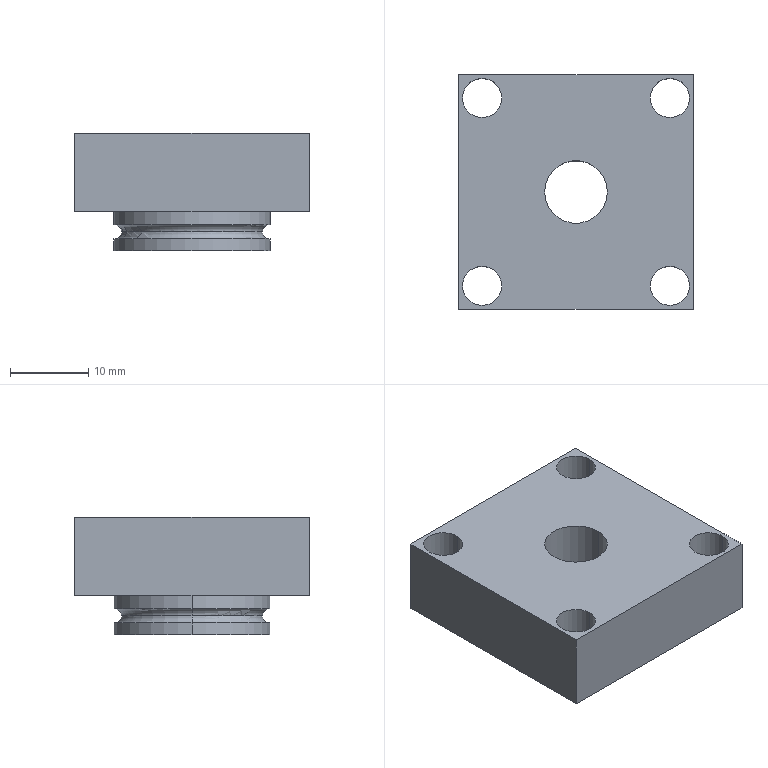Component | SolidWorks | FrontEndCapAssembly-1_CylinderFrontCover-1 | 1 solid | 25 faces | box 30 x 30 x 15 mm | volume 8944 mm3 | cylinder 14 | plane 7 | torus 4 | commonest cylinder face diameters 5 x8 20 x4 8 x2
build123d program:
from build123d import *

# Parameters (mm, degrees)
SKETCH1_W         = 30
SKETCH1_H         = 30
EXTRUDE1_DEPTH    = 10
SKETCH5_R         = 10
EXTRUDE5_DEPTH    = 5
SKETCH6_R         = 4
EXTRUDE6_DEPTH    = 30.059
SKETCH7_R         = 2.5
EXTRUDE7_DEPTH    = 30.059
CIRPATTERN1_COUNT = 4
SKETCH8_R         = 0.9


with BuildPart() as part:
    # Sketch1 → Extrude1 (new body)
    with BuildSketch(Plane.XY):
        with Locations((-3.842, -1.261)):
            Rectangle(SKETCH1_W, SKETCH1_H)
    extrude(amount=EXTRUDE1_DEPTH)

    # Sketch5 → Extrude5 (add)
    with BuildSketch(Plane.XY.offset(10)):
        with Locations((-3.842, -1.261)):
            Circle(SKETCH5_R)
    extrude(amount=EXTRUDE5_DEPTH)

    # Sketch6 → Extrude6 (cut, through all)
    with BuildSketch(Plane.XY.offset(15)):
        with Locations((-3.842, -1.261)):
            Circle(SKETCH6_R)
    extrude(amount=-EXTRUDE6_DEPTH, mode=Mode.SUBTRACT)

    # Sketch7 → Extrude7 (cut, through all)
    with BuildSketch(Plane(origin=(0, 0, 0), x_dir=(-1, 0, 0), z_dir=(0, 0, -1))):
        with Locations((-8.158, 10.739)):
            Circle(SKETCH7_R)
    extrude7 = extrude(amount=-EXTRUDE7_DEPTH, mode=Mode.SUBTRACT)

    # CirPattern1: Extrude7 ×4 about axis
    cirpattern1_axis = Axis((-3.842, -1.261, 0), (0, 0, 1))
    for i in range(1, CIRPATTERN1_COUNT):
        add(extrude7.rotate(cirpattern1_axis, i * 360 / CIRPATTERN1_COUNT), mode=Mode.SUBTRACT)

    # Sketch8 → Cut-Revolve1 (revolve, cut)
    with BuildSketch(Plane.ZY.offset(3.842), mode=Mode.PRIVATE) as cut_revolve1_sk:
        with Locations((12.6, 8.639)):
            Circle(SKETCH8_R)
    revolve(cut_revolve1_sk.sketch.rotate(Axis((-3.842, -1.261, 0), (0, 0, 1)), 90), axis=Axis((-3.842, -1.261, 0), (0, 0, 1)), mode=Mode.SUBTRACT)


solid = part.part

# Placed as in the assembly
solid = solid.moved(Location((9.967, -2.907, 52.5), (180, 0, 0)))
STEP:
#1=COLOUR_RGB('',0.7922,0.8196,0.9333);
#2=FILL_AREA_STYLE_COLOUR('',#1);
#3=FILL_AREA_STYLE('',(#2));
#4=SURFACE_STYLE_FILL_AREA(#3);
#5=SURFACE_SIDE_STYLE('',(#4));
#6=SURFACE_STYLE_USAGE(.BOTH.,#5);
#7=PRESENTATION_STYLE_ASSIGNMENT((#6));
#8=CARTESIAN_POINT('',(0.6348,-0.06482,1.606));
#9=VERTEX_POINT('',#8);
#10=CARTESIAN_POINT('',(0.5955,-0.06482,1.571));
#11=VERTEX_POINT('',#10);
#12=CARTESIAN_POINT('',(0.6309,-0.06482,1.571));
#13=DIRECTION('',(0.,-1.,-0.));
#14=DIRECTION('',(1.,0.,0.));
#15=AXIS2_PLACEMENT_3D('',#12,#13,#14);
#16=CIRCLE('',#15,0.03543);
#17=EDGE_CURVE('',#9,#11,#16,.T.);
#18=ORIENTED_EDGE('',*,*,#17,.T.);
#19=CARTESIAN_POINT('',(-0.1132,-0.06482,1.571));
#20=VERTEX_POINT('',#19);
#21=CARTESIAN_POINT('',(0.2411,-0.06482,1.571));
#22=DIRECTION('',(-0.,-0.,1.));
#23=DIRECTION('',(1.,0.,0.));
#24=AXIS2_PLACEMENT_3D('',#21,#22,#23);
#25=CIRCLE('',#24,0.3543);
#26=EDGE_CURVE('',#11,#20,#25,.T.);
#27=ORIENTED_EDGE('',*,*,#26,.T.);
#28=CARTESIAN_POINT('',(-0.1526,-0.06482,1.606));
#29=VERTEX_POINT('',#28);
#30=CARTESIAN_POINT('',(-0.1486,-0.06482,1.571));
#31=DIRECTION('',(-0.,1.,0.));
#32=DIRECTION('',(-1.,-0.,0.));
#33=AXIS2_PLACEMENT_3D('',#30,#31,#32);
#34=CIRCLE('',#33,0.03543);
#35=EDGE_CURVE('',#29,#20,#34,.T.);
#36=ORIENTED_EDGE('',*,*,#35,.F.);
#37=CARTESIAN_POINT('',(0.2411,-0.06482,1.606));
#38=DIRECTION('',(0.,0.,-1.));
#39=DIRECTION('',(-1.,-0.,0.));
#40=AXIS2_PLACEMENT_3D('',#37,#38,#39);
#41=CIRCLE('',#40,0.3937);
#42=EDGE_CURVE('',#29,#9,#41,.T.);
#43=ORIENTED_EDGE('',*,*,#42,.T.);
#44=EDGE_LOOP('',(#18,#27,#36,#43));
#45=FACE_OUTER_BOUND('',#44,.T.);
#46=CARTESIAN_POINT('',(0.2411,-0.06482,1.571));
#47=DIRECTION('',(-0.,-0.,1.));
#48=DIRECTION('',(1.,0.,0.));
#49=AXIS2_PLACEMENT_3D('',#46,#47,#48);
#50=TOROIDAL_SURFACE('',#49,0.3898,0.03543);
#51=ADVANCED_FACE('',(#45),#50,.F.);
#52=ORIENTED_EDGE('',*,*,#35,.T.);
#53=CARTESIAN_POINT('',(0.2411,-0.06482,1.571));
#54=DIRECTION('',(-0.,-0.,1.));
#55=DIRECTION('',(1.,0.,0.));
#56=AXIS2_PLACEMENT_3D('',#53,#54,#55);
#57=CIRCLE('',#56,0.3543);
#58=EDGE_CURVE('',#20,#11,#57,.T.);
#59=ORIENTED_EDGE('',*,*,#58,.T.);
#60=ORIENTED_EDGE('',*,*,#17,.F.);
#61=CARTESIAN_POINT('',(0.2411,-0.06482,1.606));
#62=DIRECTION('',(0.,0.,-1.));
#63=DIRECTION('',(-1.,-0.,0.));
#64=AXIS2_PLACEMENT_3D('',#61,#62,#63);
#65=CIRCLE('',#64,0.3937);
#66=EDGE_CURVE('',#9,#29,#65,.T.);
#67=ORIENTED_EDGE('',*,*,#66,.T.);
#68=EDGE_LOOP('',(#52,#59,#60,#67));
#69=FACE_OUTER_BOUND('',#68,.T.);
#70=CARTESIAN_POINT('',(0.2411,-0.06482,1.571));
#71=DIRECTION('',(-0.,-0.,1.));
#72=DIRECTION('',(1.,0.,0.));
#73=AXIS2_PLACEMENT_3D('',#70,#71,#72);
#74=TOROIDAL_SURFACE('',#73,0.3898,0.03543);
#75=ADVANCED_FACE('',(#69),#74,.F.);
#76=ORIENTED_EDGE('',*,*,#58,.F.);
#77=CARTESIAN_POINT('',(-0.1526,-0.06482,1.536));
#78=VERTEX_POINT('',#77);
#79=CARTESIAN_POINT('',(-0.1486,-0.06482,1.571));
#80=DIRECTION('',(-0.,1.,0.));
#81=DIRECTION('',(-1.,-0.,0.));
#82=AXIS2_PLACEMENT_3D('',#79,#80,#81);
#83=CIRCLE('',#82,0.03543);
#84=EDGE_CURVE('',#20,#78,#83,.T.);
#85=ORIENTED_EDGE('',*,*,#84,.T.);
#86=CARTESIAN_POINT('',(0.6348,-0.06482,1.536));
#87=VERTEX_POINT('',#86);
#88=CARTESIAN_POINT('',(0.2411,-0.06482,1.536));
#89=DIRECTION('',(-0.,-0.,1.));
#90=DIRECTION('',(1.,0.,0.));
#91=AXIS2_PLACEMENT_3D('',#88,#89,#90);
#92=CIRCLE('',#91,0.3937);
#93=EDGE_CURVE('',#78,#87,#92,.T.);
#94=ORIENTED_EDGE('',*,*,#93,.T.);
#95=CARTESIAN_POINT('',(0.6309,-0.06482,1.571));
#96=DIRECTION('',(0.,-1.,-0.));
#97=DIRECTION('',(1.,0.,0.));
#98=AXIS2_PLACEMENT_3D('',#95,#96,#97);
#99=CIRCLE('',#98,0.03543);
#100=EDGE_CURVE('',#11,#87,#99,.T.);
#101=ORIENTED_EDGE('',*,*,#100,.F.);
#102=EDGE_LOOP('',(#76,#85,#94,#101));
#103=FACE_OUTER_BOUND('',#102,.T.);
#104=CARTESIAN_POINT('',(0.2411,-0.06482,1.571));
#105=DIRECTION('',(-0.,-0.,1.));
#106=DIRECTION('',(1.,0.,0.));
#107=AXIS2_PLACEMENT_3D('',#104,#105,#106);
#108=TOROIDAL_SURFACE('',#107,0.3898,0.03543);
#109=ADVANCED_FACE('',(#103),#108,.F.);
#110=CARTESIAN_POINT('',(-0.1329,-0.5373,1.673));
#111=VERTEX_POINT('',#110);
#112=CARTESIAN_POINT('',(-0.3297,-0.5373,1.673));
#113=VERTEX_POINT('',#112);
#114=CARTESIAN_POINT('',(-0.2313,-0.5373,1.673));
#115=DIRECTION('',(0.,0.,-1.));
#116=DIRECTION('',(-1.,-0.,0.));
#117=AXIS2_PLACEMENT_3D('',#114,#115,#116);
#118=CIRCLE('',#117,0.09843);
#119=EDGE_CURVE('',#111,#113,#118,.T.);
#120=ORIENTED_EDGE('',*,*,#119,.T.);
#121=CARTESIAN_POINT('',(-0.3297,-0.5373,2.067));
#122=VERTEX_POINT('',#121);
#123=CARTESIAN_POINT('',(-0.3297,-0.5373,1.476));
#124=DIRECTION('',(-0.,-0.,1.));
#125=VECTOR('',#124,39.37);
#126=LINE('',#123,#125);
#127=EDGE_CURVE('',#113,#122,#126,.T.);
#128=ORIENTED_EDGE('',*,*,#127,.T.);
#129=CARTESIAN_POINT('',(-0.1329,-0.5373,2.067));
#130=VERTEX_POINT('',#129);
#131=CARTESIAN_POINT('',(-0.2313,-0.5373,2.067));
#132=DIRECTION('',(-0.,-0.,1.));
#133=DIRECTION('',(0.,1.,0.));
#134=AXIS2_PLACEMENT_3D('',#131,#132,#133);
#135=CIRCLE('',#134,0.09843);
#136=EDGE_CURVE('',#122,#130,#135,.T.);
#137=ORIENTED_EDGE('',*,*,#136,.T.);
#138=CARTESIAN_POINT('',(-0.1329,-0.5373,1.476));
#139=DIRECTION('',(-0.,-0.,1.));
#140=VECTOR('',#139,39.37);
#141=LINE('',#138,#140);
#142=EDGE_CURVE('',#111,#130,#141,.T.);
#143=ORIENTED_EDGE('',*,*,#142,.F.);
#144=EDGE_LOOP('',(#120,#128,#137,#143));
#145=FACE_OUTER_BOUND('',#144,.T.);
#146=CARTESIAN_POINT('',(-0.2313,-0.5373,1.476));
#147=DIRECTION('',(-0.,-0.,1.));
#148=DIRECTION('',(1.,0.,0.));
#149=AXIS2_PLACEMENT_3D('',#146,#147,#148);
#150=CYLINDRICAL_SURFACE('',#149,0.09843);
#151=ADVANCED_FACE('',(#145),#150,.F.);
#152=CARTESIAN_POINT('',(0.812,-0.5373,1.673));
#153=VERTEX_POINT('',#152);
#154=CARTESIAN_POINT('',(0.6152,-0.5373,1.673));
#155=VERTEX_POINT('',#154);
#156=CARTESIAN_POINT('',(0.7136,-0.5373,1.673));
#157=DIRECTION('',(0.,0.,-1.));
#158=DIRECTION('',(-1.,-0.,0.));
#159=AXIS2_PLACEMENT_3D('',#156,#157,#158);
#160=CIRCLE('',#159,0.09843);
#161=EDGE_CURVE('',#153,#155,#160,.T.);
#162=ORIENTED_EDGE('',*,*,#161,.T.);
#163=CARTESIAN_POINT('',(0.6152,-0.5373,2.067));
#164=VERTEX_POINT('',#163);
#165=CARTESIAN_POINT('',(0.6152,-0.5373,1.476));
#166=DIRECTION('',(-0.,-0.,1.));
#167=VECTOR('',#166,39.37);
#168=LINE('',#165,#167);
#169=EDGE_CURVE('',#155,#164,#168,.T.);
#170=ORIENTED_EDGE('',*,*,#169,.T.);
#171=CARTESIAN_POINT('',(0.812,-0.5373,2.067));
#172=VERTEX_POINT('',#171);
#173=CARTESIAN_POINT('',(0.7136,-0.5373,2.067));
#174=DIRECTION('',(-0.,-0.,1.));
#175=DIRECTION('',(-1.,0.,0.));
#176=AXIS2_PLACEMENT_3D('',#173,#174,#175);
#177=CIRCLE('',#176,0.09843);
#178=EDGE_CURVE('',#164,#172,#177,.T.);
#179=ORIENTED_EDGE('',*,*,#178,.T.);
#180=CARTESIAN_POINT('',(0.812,-0.5373,1.476));
#181=DIRECTION('',(-0.,-0.,1.));
#182=VECTOR('',#181,39.37);
#183=LINE('',#180,#182);
#184=EDGE_CURVE('',#153,#172,#183,.T.);
#185=ORIENTED_EDGE('',*,*,#184,.F.);
#186=EDGE_LOOP('',(#162,#170,#179,#185));
#187=FACE_OUTER_BOUND('',#186,.T.);
#188=CARTESIAN_POINT('',(0.7136,-0.5373,1.476));
#189=DIRECTION('',(-0.,-0.,1.));
#190=DIRECTION('',(1.,0.,0.));
#191=AXIS2_PLACEMENT_3D('',#188,#189,#190);
#192=CYLINDRICAL_SURFACE('',#191,0.09843);
#193=ADVANCED_FACE('',(#187),#192,.F.);
#194=CARTESIAN_POINT('',(0.812,0.4076,1.673));
#195=VERTEX_POINT('',#194);
#196=CARTESIAN_POINT('',(0.6152,0.4076,1.673));
#197=VERTEX_POINT('',#196);
#198=CARTESIAN_POINT('',(0.7136,0.4076,1.673));
#199=DIRECTION('',(0.,0.,-1.));
#200=DIRECTION('',(-1.,-0.,0.));
#201=AXIS2_PLACEMENT_3D('',#198,#199,#200);
#202=CIRCLE('',#201,0.09843);
#203=EDGE_CURVE('',#195,#197,#202,.T.);
#204=ORIENTED_EDGE('',*,*,#203,.T.);
#205=CARTESIAN_POINT('',(0.6152,0.4076,2.067));
#206=VERTEX_POINT('',#205);
#207=CARTESIAN_POINT('',(0.6152,0.4076,1.476));
#208=DIRECTION('',(-0.,-0.,1.));
#209=VECTOR('',#208,39.37);
#210=LINE('',#207,#209);
#211=EDGE_CURVE('',#197,#206,#210,.T.);
#212=ORIENTED_EDGE('',*,*,#211,.T.);
#213=CARTESIAN_POINT('',(0.812,0.4076,2.067));
#214=VERTEX_POINT('',#213);
#215=CARTESIAN_POINT('',(0.7136,0.4076,2.067));
#216=DIRECTION('',(-0.,-0.,1.));
#217=DIRECTION('',(-0.,-1.,0.));
#218=AXIS2_PLACEMENT_3D('',#215,#216,#217);
#219=CIRCLE('',#218,0.09843);
#220=EDGE_CURVE('',#206,#214,#219,.T.);
#221=ORIENTED_EDGE('',*,*,#220,.T.);
#222=CARTESIAN_POINT('',(0.812,0.4076,1.476));
#223=DIRECTION('',(-0.,-0.,1.));
#224=VECTOR('',#223,39.37);
#225=LINE('',#222,#224);
#226=EDGE_CURVE('',#195,#214,#225,.T.);
#227=ORIENTED_EDGE('',*,*,#226,.F.);
#228=EDGE_LOOP('',(#204,#212,#221,#227));
#229=FACE_OUTER_BOUND('',#228,.T.);
#230=CARTESIAN_POINT('',(0.7136,0.4076,1.476));
#231=DIRECTION('',(-0.,-0.,1.));
#232=DIRECTION('',(1.,0.,0.));
#233=AXIS2_PLACEMENT_3D('',#230,#231,#232);
#234=CYLINDRICAL_SURFACE('',#233,0.09843);
#235=ADVANCED_FACE('',(#229),#234,.F.);
#236=CARTESIAN_POINT('',(-0.1329,0.4076,1.673));
#237=VERTEX_POINT('',#236);
#238=CARTESIAN_POINT('',(-0.3297,0.4076,1.673));
#239=VERTEX_POINT('',#238);
#240=CARTESIAN_POINT('',(-0.2313,0.4076,1.673));
#241=DIRECTION('',(0.,0.,-1.));
#242=DIRECTION('',(-1.,-0.,0.));
#243=AXIS2_PLACEMENT_3D('',#240,#241,#242);
#244=CIRCLE('',#243,0.09843);
#245=EDGE_CURVE('',#237,#239,#244,.T.);
#246=ORIENTED_EDGE('',*,*,#245,.T.);
#247=CARTESIAN_POINT('',(-0.3297,0.4076,2.067));
#248=VERTEX_POINT('',#247);
#249=CARTESIAN_POINT('',(-0.3297,0.4076,1.476));
#250=DIRECTION('',(-0.,-0.,1.));
#251=VECTOR('',#250,39.37);
#252=LINE('',#249,#251);
#253=EDGE_CURVE('',#239,#248,#252,.T.);
#254=ORIENTED_EDGE('',*,*,#253,.T.);
#255=CARTESIAN_POINT('',(-0.1329,0.4076,2.067));
#256=VERTEX_POINT('',#255);
#257=CARTESIAN_POINT('',(-0.2313,0.4076,2.067));
#258=DIRECTION('',(-0.,-0.,1.));
#259=DIRECTION('',(1.,0.,0.));
#260=AXIS2_PLACEMENT_3D('',#257,#258,#259);
#261=CIRCLE('',#260,0.09843);
#262=EDGE_CURVE('',#248,#256,#261,.T.);
#263=ORIENTED_EDGE('',*,*,#262,.T.);
#264=CARTESIAN_POINT('',(-0.1329,0.4076,1.476));
#265=DIRECTION('',(-0.,-0.,1.));
#266=VECTOR('',#265,39.37);
#267=LINE('',#264,#266);
#268=EDGE_CURVE('',#237,#256,#267,.T.);
#269=ORIENTED_EDGE('',*,*,#268,.F.);
#270=EDGE_LOOP('',(#246,#254,#263,#269));
#271=FACE_OUTER_BOUND('',#270,.T.);
#272=CARTESIAN_POINT('',(-0.2313,0.4076,1.476));
#273=DIRECTION('',(-0.,-0.,1.));
#274=DIRECTION('',(1.,0.,0.));
#275=AXIS2_PLACEMENT_3D('',#272,#273,#274);
#276=CYLINDRICAL_SURFACE('',#275,0.09843);
#277=ADVANCED_FACE('',(#271),#276,.F.);
#278=CARTESIAN_POINT('',(0.3986,-0.06482,2.067));
#279=VERTEX_POINT('',#278);
#280=CARTESIAN_POINT('',(0.08366,-0.06482,2.067));
#281=VERTEX_POINT('',#280);
#282=CARTESIAN_POINT('',(0.2411,-0.06482,2.067));
#283=DIRECTION('',(0.,0.,-1.));
#284=DIRECTION('',(-1.,-0.,0.));
#285=AXIS2_PLACEMENT_3D('',#282,#283,#284);
#286=CIRCLE('',#285,0.1575);
#287=EDGE_CURVE('',#279,#281,#286,.T.);
#288=ORIENTED_EDGE('',*,*,#287,.F.);
#289=CARTESIAN_POINT('',(0.3986,-0.06482,1.476));
#290=VERTEX_POINT('',#289);
#291=CARTESIAN_POINT('',(0.3986,-0.06482,2.067));
#292=DIRECTION('',(0.,0.,-1.));
#293=VECTOR('',#292,39.37);
#294=LINE('',#291,#293);
#295=EDGE_CURVE('',#279,#290,#294,.T.);
#296=ORIENTED_EDGE('',*,*,#295,.T.);
#297=CARTESIAN_POINT('',(0.08366,-0.06482,1.476));
#298=VERTEX_POINT('',#297);
#299=CARTESIAN_POINT('',(0.2411,-0.06482,1.476));
#300=DIRECTION('',(0.,0.,-1.));
#301=DIRECTION('',(-1.,-0.,0.));
#302=AXIS2_PLACEMENT_3D('',#299,#300,#301);
#303=CIRCLE('',#302,0.1575);
#304=EDGE_CURVE('',#290,#298,#303,.T.);
#305=ORIENTED_EDGE('',*,*,#304,.T.);
#306=CARTESIAN_POINT('',(0.08366,-0.06482,2.067));
#307=DIRECTION('',(0.,0.,-1.));
#308=VECTOR('',#307,39.37);
#309=LINE('',#306,#308);
#310=EDGE_CURVE('',#281,#298,#309,.T.);
#311=ORIENTED_EDGE('',*,*,#310,.F.);
#312=EDGE_LOOP('',(#288,#296,#305,#311));
#313=FACE_OUTER_BOUND('',#312,.T.);
#314=CARTESIAN_POINT('',(0.2411,-0.06482,2.067));
#315=DIRECTION('',(0.,0.,-1.));
#316=DIRECTION('',(-1.,-0.,0.));
#317=AXIS2_PLACEMENT_3D('',#314,#315,#316);
#318=CYLINDRICAL_SURFACE('',#317,0.1575);
#319=ADVANCED_FACE('',(#313),#318,.F.);
#320=CARTESIAN_POINT('',(-0.1526,-0.06482,1.476));
#321=VERTEX_POINT('',#320);
#322=CARTESIAN_POINT('',(0.6348,-0.06482,1.476));
#323=VERTEX_POINT('',#322);
#324=CARTESIAN_POINT('',(0.2411,-0.06482,1.476));
#325=DIRECTION('',(0.,0.,-1.));
#326=DIRECTION('',(-1.,-0.,0.));
#327=AXIS2_PLACEMENT_3D('',#324,#325,#326);
#328=CIRCLE('',#327,0.3937);
#329=EDGE_CURVE('',#321,#323,#328,.T.);
#330=ORIENTED_EDGE('',*,*,#329,.F.);
#331=CARTESIAN_POINT('',(-0.1526,-0.06482,1.476));
#332=DIRECTION('',(-0.,-0.,1.));
#333=VECTOR('',#332,39.37);
#334=LINE('',#331,#333);
#335=EDGE_CURVE('',#321,#78,#334,.T.);
#336=ORIENTED_EDGE('',*,*,#335,.T.);
#337=CARTESIAN_POINT('',(0.2411,-0.06482,1.536));
#338=DIRECTION('',(-0.,-0.,1.));
#339=DIRECTION('',(1.,0.,0.));
#340=AXIS2_PLACEMENT_3D('',#337,#338,#339);
#341=CIRCLE('',#340,0.3937);
#342=EDGE_CURVE('',#87,#78,#341,.T.);
#343=ORIENTED_EDGE('',*,*,#342,.F.);
#344=CARTESIAN_POINT('',(0.6348,-0.06482,1.476));
#345=DIRECTION('',(-0.,-0.,1.));
#346=VECTOR('',#345,39.37);
#347=LINE('',#344,#346);
#348=EDGE_CURVE('',#323,#87,#347,.T.);
#349=ORIENTED_EDGE('',*,*,#348,.F.);
#350=EDGE_LOOP('',(#330,#336,#343,#349));
#351=FACE_OUTER_BOUND('',#350,.T.);
#352=CARTESIAN_POINT('',(0.2411,-0.06482,1.476));
#353=DIRECTION('',(-0.,-0.,1.));
#354=DIRECTION('',(1.,0.,0.));
#355=AXIS2_PLACEMENT_3D('',#352,#353,#354);
#356=CYLINDRICAL_SURFACE('',#355,0.3937);
#357=ADVANCED_FACE('',(#351),#356,.T.);
#358=ORIENTED_EDGE('',*,*,#42,.F.);
#359=CARTESIAN_POINT('',(-0.1526,-0.06482,1.673));
#360=VERTEX_POINT('',#359);
#361=CARTESIAN_POINT('',(-0.1526,-0.06482,1.476));
#362=DIRECTION('',(-0.,-0.,1.));
#363=VECTOR('',#362,39.37);
#364=LINE('',#361,#363);
#365=EDGE_CURVE('',#29,#360,#364,.T.);
#366=ORIENTED_EDGE('',*,*,#365,.T.);
#367=CARTESIAN_POINT('',(0.6348,-0.06482,1.673));
#368=VERTEX_POINT('',#367);
#369=CARTESIAN_POINT('',(0.2411,-0.06482,1.673));
#370=DIRECTION('',(0.,0.,-1.));
#371=DIRECTION('',(-1.,-0.,0.));
#372=AXIS2_PLACEMENT_3D('',#369,#370,#371);
#373=CIRCLE('',#372,0.3937);
#374=EDGE_CURVE('',#360,#368,#373,.T.);
#375=ORIENTED_EDGE('',*,*,#374,.T.);
#376=CARTESIAN_POINT('',(0.6348,-0.06482,1.476));
#377=DIRECTION('',(-0.,-0.,1.));
#378=VECTOR('',#377,39.37);
#379=LINE('',#376,#378);
#380=EDGE_CURVE('',#9,#368,#379,.T.);
#381=ORIENTED_EDGE('',*,*,#380,.F.);
#382=EDGE_LOOP('',(#358,#366,#375,#381));
#383=FACE_OUTER_BOUND('',#382,.T.);
#384=CARTESIAN_POINT('',(0.2411,-0.06482,1.476));
#385=DIRECTION('',(-0.,-0.,1.));
#386=DIRECTION('',(1.,0.,0.));
#387=AXIS2_PLACEMENT_3D('',#384,#385,#386);
#388=CYLINDRICAL_SURFACE('',#387,0.3937);
#389=ADVANCED_FACE('',(#383),#388,.T.);
#390=ORIENTED_EDGE('',*,*,#365,.F.);
#391=ORIENTED_EDGE('',*,*,#66,.F.);
#392=ORIENTED_EDGE('',*,*,#380,.T.);
#393=CARTESIAN_POINT('',(0.2411,-0.06482,1.673));
#394=DIRECTION('',(0.,0.,-1.));
#395=DIRECTION('',(-1.,-0.,0.));
#396=AXIS2_PLACEMENT_3D('',#393,#394,#395);
#397=CIRCLE('',#396,0.3937);
#398=EDGE_CURVE('',#368,#360,#397,.T.);
#399=ORIENTED_EDGE('',*,*,#398,.T.);
#400=EDGE_LOOP('',(#390,#391,#392,#399));
#401=FACE_OUTER_BOUND('',#400,.T.);
#402=CARTESIAN_POINT('',(0.2411,-0.06482,1.476));
#403=DIRECTION('',(-0.,-0.,1.));
#404=DIRECTION('',(1.,0.,0.));
#405=AXIS2_PLACEMENT_3D('',#402,#403,#404);
#406=CYLINDRICAL_SURFACE('',#405,0.3937);
#407=ADVANCED_FACE('',(#401),#406,.T.);
#408=ORIENTED_EDGE('',*,*,#335,.F.);
#409=CARTESIAN_POINT('',(0.2411,-0.06482,1.476));
#410=DIRECTION('',(0.,0.,-1.));
#411=DIRECTION('',(-1.,-0.,0.));
#412=AXIS2_PLACEMENT_3D('',#409,#410,#411);
#413=CIRCLE('',#412,0.3937);
#414=EDGE_CURVE('',#323,#321,#413,.T.);
#415=ORIENTED_EDGE('',*,*,#414,.F.);
#416=ORIENTED_EDGE('',*,*,#348,.T.);
#417=ORIENTED_EDGE('',*,*,#93,.F.);
#418=EDGE_LOOP('',(#408,#415,#416,#417));
#419=FACE_OUTER_BOUND('',#418,.T.);
#420=CARTESIAN_POINT('',(0.2411,-0.06482,1.476));
#421=DIRECTION('',(-0.,-0.,1.));
#422=DIRECTION('',(1.,0.,0.));
#423=AXIS2_PLACEMENT_3D('',#420,#421,#422);
#424=CYLINDRICAL_SURFACE('',#423,0.3937);
#425=ADVANCED_FACE('',(#419),#424,.T.);
#426=ORIENTED_EDGE('',*,*,#119,.F.);
#427=CARTESIAN_POINT('',(-0.2313,-0.5373,1.673));
#428=DIRECTION('',(0.,0.,-1.));
#429=DIRECTION('',(-1.,-0.,0.));
#430=AXIS2_PLACEMENT_3D('',#427,#428,#429);
#431=CIRCLE('',#430,0.09843);
#432=EDGE_CURVE('',#113,#111,#431,.T.);
#433=ORIENTED_EDGE('',*,*,#432,.F.);
#434=EDGE_LOOP('',(#426,#433));
#435=FACE_BOUND('',#434,.T.);
#436=ORIENTED_EDGE('',*,*,#161,.F.);
#437=CARTESIAN_POINT('',(0.7136,-0.5373,1.673));
#438=DIRECTION('',(0.,0.,-1.));
#439=DIRECTION('',(-1.,-0.,0.));
#440=AXIS2_PLACEMENT_3D('',#437,#438,#439);
#441=CIRCLE('',#440,0.09843);
#442=EDGE_CURVE('',#155,#153,#441,.T.);
#443=ORIENTED_EDGE('',*,*,#442,.F.);
#444=EDGE_LOOP('',(#436,#443));
#445=FACE_BOUND('',#444,.T.);
#446=ORIENTED_EDGE('',*,*,#203,.F.);
#447=CARTESIAN_POINT('',(0.7136,0.4076,1.673));
#448=DIRECTION('',(0.,0.,-1.));
#449=DIRECTION('',(-1.,-0.,0.));
#450=AXIS2_PLACEMENT_3D('',#447,#448,#449);
#451=CIRCLE('',#450,0.09843);
#452=EDGE_CURVE('',#197,#195,#451,.T.);
#453=ORIENTED_EDGE('',*,*,#452,.F.);
#454=EDGE_LOOP('',(#446,#453));
#455=FACE_BOUND('',#454,.T.);
#456=ORIENTED_EDGE('',*,*,#245,.F.);
#457=CARTESIAN_POINT('',(-0.2313,0.4076,1.673));
#458=DIRECTION('',(0.,0.,-1.));
#459=DIRECTION('',(-1.,-0.,0.));
#460=AXIS2_PLACEMENT_3D('',#457,#458,#459);
#461=CIRCLE('',#460,0.09843);
#462=EDGE_CURVE('',#239,#237,#461,.T.);
#463=ORIENTED_EDGE('',*,*,#462,.F.);
#464=EDGE_LOOP('',(#456,#463));
#465=FACE_BOUND('',#464,.T.);
#466=CARTESIAN_POINT('',(0.8317,0.5257,1.673));
#467=VERTEX_POINT('',#466);
#468=CARTESIAN_POINT('',(0.8317,-0.6554,1.673));
#469=VERTEX_POINT('',#468);
#470=CARTESIAN_POINT('',(0.8317,0.5257,1.673));
#471=DIRECTION('',(0.,-1.,-0.));
#472=VECTOR('',#471,39.37);
#473=LINE('',#470,#472);
#474=EDGE_CURVE('',#467,#469,#473,.T.);
#475=ORIENTED_EDGE('',*,*,#474,.T.);
#476=CARTESIAN_POINT('',(-0.3494,-0.6554,1.673));
#477=VERTEX_POINT('',#476);
#478=CARTESIAN_POINT('',(0.8317,-0.6554,1.673));
#479=DIRECTION('',(-1.,-0.,-0.));
#480=VECTOR('',#479,39.37);
#481=LINE('',#478,#480);
#482=EDGE_CURVE('',#469,#477,#481,.T.);
#483=ORIENTED_EDGE('',*,*,#482,.T.);
#484=CARTESIAN_POINT('',(-0.3494,0.5257,1.673));
#485=VERTEX_POINT('',#484);
#486=CARTESIAN_POINT('',(-0.3494,0.5257,1.673));
#487=DIRECTION('',(-0.,1.,0.));
#488=VECTOR('',#487,39.37);
#489=LINE('',#486,#488);
#490=EDGE_CURVE('',#477,#485,#489,.T.);
#491=ORIENTED_EDGE('',*,*,#490,.T.);
#492=CARTESIAN_POINT('',(0.8317,0.5257,1.673));
#493=DIRECTION('',(1.,0.,0.));
#494=VECTOR('',#493,39.37);
#495=LINE('',#492,#494);
#496=EDGE_CURVE('',#485,#467,#495,.T.);
#497=ORIENTED_EDGE('',*,*,#496,.T.);
#498=EDGE_LOOP('',(#475,#483,#491,#497));
#499=FACE_OUTER_BOUND('',#498,.T.);
#500=ORIENTED_EDGE('',*,*,#398,.F.);
#501=ORIENTED_EDGE('',*,*,#374,.F.);
#502=EDGE_LOOP('',(#500,#501));
#503=FACE_BOUND('',#502,.T.);
#504=CARTESIAN_POINT('',(0.8317,-0.6554,1.673));
#505=DIRECTION('',(0.,0.,-1.));
#506=DIRECTION('',(-1.,-0.,-0.));
#507=AXIS2_PLACEMENT_3D('',#504,#505,#506);
#508=PLANE('',#507);
#509=ADVANCED_FACE('',(#435,#445,#455,#465,#499,#503),#508,.T.);
#510=CARTESIAN_POINT('',(0.8317,0.5257,2.067));
#511=VERTEX_POINT('',#510);
#512=CARTESIAN_POINT('',(0.8317,-0.6554,2.067));
#513=VERTEX_POINT('',#512);
#514=CARTESIAN_POINT('',(0.8317,0.5257,2.067));
#515=DIRECTION('',(0.,-1.,-0.));
#516=VECTOR('',#515,39.37);
#517=LINE('',#514,#516);
#518=EDGE_CURVE('',#511,#513,#517,.T.);
#519=ORIENTED_EDGE('',*,*,#518,.T.);
#520=CARTESIAN_POINT('',(0.8317,-0.6554,1.673));
#521=DIRECTION('',(-0.,-0.,1.));
#522=VECTOR('',#521,39.37);
#523=LINE('',#520,#522);
#524=EDGE_CURVE('',#469,#513,#523,.T.);
#525=ORIENTED_EDGE('',*,*,#524,.F.);
#526=ORIENTED_EDGE('',*,*,#474,.F.);
#527=CARTESIAN_POINT('',(0.8317,0.5257,1.673));
#528=DIRECTION('',(-0.,-0.,1.));
#529=VECTOR('',#528,39.37);
#530=LINE('',#527,#529);
#531=EDGE_CURVE('',#467,#511,#530,.T.);
#532=ORIENTED_EDGE('',*,*,#531,.T.);
#533=EDGE_LOOP('',(#519,#525,#526,#532));
#534=FACE_OUTER_BOUND('',#533,.T.);
#535=CARTESIAN_POINT('',(0.8317,0.5257,1.673));
#536=DIRECTION('',(-1.,-0.,-0.));
#537=DIRECTION('',(-0.,-0.,1.));
#538=AXIS2_PLACEMENT_3D('',#535,#536,#537);
#539=PLANE('',#538);
#540=ADVANCED_FACE('',(#534),#539,.F.);
#541=CARTESIAN_POINT('',(-0.3494,-0.6554,2.067));
#542=VERTEX_POINT('',#541);
#543=CARTESIAN_POINT('',(0.8317,-0.6554,2.067));
#544=DIRECTION('',(-1.,-0.,-0.));
#545=VECTOR('',#544,39.37);
#546=LINE('',#543,#545);
#547=EDGE_CURVE('',#513,#542,#546,.T.);
#548=ORIENTED_EDGE('',*,*,#547,.T.);
#549=CARTESIAN_POINT('',(-0.3494,-0.6554,1.673));
#550=DIRECTION('',(-0.,-0.,1.));
#551=VECTOR('',#550,39.37);
#552=LINE('',#549,#551);
#553=EDGE_CURVE('',#477,#542,#552,.T.);
#554=ORIENTED_EDGE('',*,*,#553,.F.);
#555=ORIENTED_EDGE('',*,*,#482,.F.);
#556=ORIENTED_EDGE('',*,*,#524,.T.);
#557=EDGE_LOOP('',(#548,#554,#555,#556));
#558=FACE_OUTER_BOUND('',#557,.T.);
#559=CARTESIAN_POINT('',(0.8317,-0.6554,1.673));
#560=DIRECTION('',(-0.,1.,0.));
#561=DIRECTION('',(0.,0.,-1.));
#562=AXIS2_PLACEMENT_3D('',#559,#560,#561);
#563=PLANE('',#562);
#564=ADVANCED_FACE('',(#558),#563,.F.);
#565=CARTESIAN_POINT('',(-0.3494,0.5257,2.067));
#566=VERTEX_POINT('',#565);
#567=CARTESIAN_POINT('',(-0.3494,0.5257,2.067));
#568=DIRECTION('',(-0.,1.,0.));
#569=VECTOR('',#568,39.37);
#570=LINE('',#567,#569);
#571=EDGE_CURVE('',#542,#566,#570,.T.);
#572=ORIENTED_EDGE('',*,*,#571,.T.);
#573=CARTESIAN_POINT('',(-0.3494,0.5257,1.673));
#574=DIRECTION('',(-0.,-0.,1.));
#575=VECTOR('',#574,39.37);
#576=LINE('',#573,#575);
#577=EDGE_CURVE('',#485,#566,#576,.T.);
#578=ORIENTED_EDGE('',*,*,#577,.F.);
#579=ORIENTED_EDGE('',*,*,#490,.F.);
#580=ORIENTED_EDGE('',*,*,#553,.T.);
#581=EDGE_LOOP('',(#572,#578,#579,#580));
#582=FACE_OUTER_BOUND('',#581,.T.);
#583=CARTESIAN_POINT('',(-0.3494,0.5257,1.673));
#584=DIRECTION('',(1.,0.,0.));
#585=DIRECTION('',(0.,-1.,-0.));
#586=AXIS2_PLACEMENT_3D('',#583,#584,#585);
#587=PLANE('',#586);
#588=ADVANCED_FACE('',(#582),#587,.F.);
#589=CARTESIAN_POINT('',(0.8317,0.5257,2.067));
#590=DIRECTION('',(1.,0.,0.));
#591=VECTOR('',#590,39.37);
#592=LINE('',#589,#591);
#593=EDGE_CURVE('',#566,#511,#592,.T.);
#594=ORIENTED_EDGE('',*,*,#593,.T.);
#595=ORIENTED_EDGE('',*,*,#531,.F.);
#596=ORIENTED_EDGE('',*,*,#496,.F.);
#597=ORIENTED_EDGE('',*,*,#577,.T.);
#598=EDGE_LOOP('',(#594,#595,#596,#597));
#599=FACE_OUTER_BOUND('',#598,.T.);
#600=CARTESIAN_POINT('',(0.8317,0.5257,1.673));
#601=DIRECTION('',(0.,-1.,-0.));
#602=DIRECTION('',(-0.,-0.,1.));
#603=AXIS2_PLACEMENT_3D('',#600,#601,#602);
#604=PLANE('',#603);
#605=ADVANCED_FACE('',(#599),#604,.F.);
#606=CARTESIAN_POINT('',(-0.2313,-0.5373,2.067));
#607=DIRECTION('',(-0.,-0.,1.));
#608=DIRECTION('',(0.,1.,0.));
#609=AXIS2_PLACEMENT_3D('',#606,#607,#608);
#610=CIRCLE('',#609,0.09843);
#611=EDGE_CURVE('',#130,#122,#610,.T.);
#612=ORIENTED_EDGE('',*,*,#611,.F.);
#613=ORIENTED_EDGE('',*,*,#136,.F.);
#614=EDGE_LOOP('',(#612,#613));
#615=FACE_BOUND('',#614,.T.);
#616=CARTESIAN_POINT('',(0.7136,-0.5373,2.067));
#617=DIRECTION('',(-0.,-0.,1.));
#618=DIRECTION('',(-1.,0.,0.));
#619=AXIS2_PLACEMENT_3D('',#616,#617,#618);
#620=CIRCLE('',#619,0.09843);
#621=EDGE_CURVE('',#172,#164,#620,.T.);
#622=ORIENTED_EDGE('',*,*,#621,.F.);
#623=ORIENTED_EDGE('',*,*,#178,.F.);
#624=EDGE_LOOP('',(#622,#623));
#625=FACE_BOUND('',#624,.T.);
#626=CARTESIAN_POINT('',(0.7136,0.4076,2.067));
#627=DIRECTION('',(-0.,-0.,1.));
#628=DIRECTION('',(-0.,-1.,0.));
#629=AXIS2_PLACEMENT_3D('',#626,#627,#628);
#630=CIRCLE('',#629,0.09843);
#631=EDGE_CURVE('',#214,#206,#630,.T.);
#632=ORIENTED_EDGE('',*,*,#631,.F.);
#633=ORIENTED_EDGE('',*,*,#220,.F.);
#634=EDGE_LOOP('',(#632,#633));
#635=FACE_BOUND('',#634,.T.);
#636=CARTESIAN_POINT('',(-0.2313,0.4076,2.067));
#637=DIRECTION('',(-0.,-0.,1.));
#638=DIRECTION('',(1.,0.,0.));
#639=AXIS2_PLACEMENT_3D('',#636,#637,#638);
#640=CIRCLE('',#639,0.09843);
#641=EDGE_CURVE('',#256,#248,#640,.T.);
#642=ORIENTED_EDGE('',*,*,#641,.F.);
#643=ORIENTED_EDGE('',*,*,#262,.F.);
#644=EDGE_LOOP('',(#642,#643));
#645=FACE_BOUND('',#644,.T.);
#646=CARTESIAN_POINT('',(0.2411,-0.06482,2.067));
#647=DIRECTION('',(0.,0.,-1.));
#648=DIRECTION('',(-1.,-0.,0.));
#649=AXIS2_PLACEMENT_3D('',#646,#647,#648);
#650=CIRCLE('',#649,0.1575);
#651=EDGE_CURVE('',#281,#279,#650,.T.);
#652=ORIENTED_EDGE('',*,*,#651,.T.);
#653=ORIENTED_EDGE('',*,*,#287,.T.);
#654=EDGE_LOOP('',(#652,#653));
#655=FACE_BOUND('',#654,.T.);
#656=ORIENTED_EDGE('',*,*,#518,.F.);
#657=ORIENTED_EDGE('',*,*,#593,.F.);
#658=ORIENTED_EDGE('',*,*,#571,.F.);
#659=ORIENTED_EDGE('',*,*,#547,.F.);
#660=EDGE_LOOP('',(#656,#657,#658,#659));
#661=FACE_OUTER_BOUND('',#660,.T.);
#662=CARTESIAN_POINT('',(0.8317,-0.6554,2.067));
#663=DIRECTION('',(0.,0.,-1.));
#664=DIRECTION('',(-1.,-0.,-0.));
#665=AXIS2_PLACEMENT_3D('',#662,#663,#664);
#666=PLANE('',#665);
#667=ADVANCED_FACE('',(#615,#625,#635,#645,#655,#661),#666,.F.);
#668=CARTESIAN_POINT('',(0.2411,-0.06482,1.476));
#669=DIRECTION('',(0.,0.,-1.));
#670=DIRECTION('',(-1.,-0.,0.));
#671=AXIS2_PLACEMENT_3D('',#668,#669,#670);
#672=CIRCLE('',#671,0.1575);
#673=EDGE_CURVE('',#298,#290,#672,.T.);
#674=ORIENTED_EDGE('',*,*,#673,.F.);
#675=ORIENTED_EDGE('',*,*,#304,.F.);
#676=EDGE_LOOP('',(#674,#675));
#677=FACE_BOUND('',#676,.T.);
#678=ORIENTED_EDGE('',*,*,#414,.T.);
#679=ORIENTED_EDGE('',*,*,#329,.T.);
#680=EDGE_LOOP('',(#678,#679));
#681=FACE_OUTER_BOUND('',#680,.T.);
#682=CARTESIAN_POINT('',(0.2411,-0.06482,1.476));
#683=DIRECTION('',(0.,0.,-1.));
#684=DIRECTION('',(-1.,-0.,-0.));
#685=AXIS2_PLACEMENT_3D('',#682,#683,#684);
#686=PLANE('',#685);
#687=ADVANCED_FACE('',(#677,#681),#686,.T.);
#688=ORIENTED_EDGE('',*,*,#295,.F.);
#689=ORIENTED_EDGE('',*,*,#651,.F.);
#690=ORIENTED_EDGE('',*,*,#310,.T.);
#691=ORIENTED_EDGE('',*,*,#673,.T.);
#692=EDGE_LOOP('',(#688,#689,#690,#691));
#693=FACE_OUTER_BOUND('',#692,.T.);
#694=CARTESIAN_POINT('',(0.2411,-0.06482,2.067));
#695=DIRECTION('',(0.,0.,-1.));
#696=DIRECTION('',(-1.,-0.,0.));
#697=AXIS2_PLACEMENT_3D('',#694,#695,#696);
#698=CYLINDRICAL_SURFACE('',#697,0.1575);
#699=ADVANCED_FACE('',(#693),#698,.F.);
#700=ORIENTED_EDGE('',*,*,#253,.F.);
#701=ORIENTED_EDGE('',*,*,#462,.T.);
#702=ORIENTED_EDGE('',*,*,#268,.T.);
#703=ORIENTED_EDGE('',*,*,#641,.T.);
#704=EDGE_LOOP('',(#700,#701,#702,#703));
#705=FACE_OUTER_BOUND('',#704,.T.);
#706=CARTESIAN_POINT('',(-0.2313,0.4076,1.476));
#707=DIRECTION('',(-0.,-0.,1.));
#708=DIRECTION('',(1.,0.,0.));
#709=AXIS2_PLACEMENT_3D('',#706,#707,#708);
#710=CYLINDRICAL_SURFACE('',#709,0.09843);
#711=ADVANCED_FACE('',(#705),#710,.F.);
#712=ORIENTED_EDGE('',*,*,#211,.F.);
#713=ORIENTED_EDGE('',*,*,#452,.T.);
#714=ORIENTED_EDGE('',*,*,#226,.T.);
#715=ORIENTED_EDGE('',*,*,#631,.T.);
#716=EDGE_LOOP('',(#712,#713,#714,#715));
#717=FACE_OUTER_BOUND('',#716,.T.);
#718=CARTESIAN_POINT('',(0.7136,0.4076,1.476));
#719=DIRECTION('',(-0.,-0.,1.));
#720=DIRECTION('',(1.,0.,0.));
#721=AXIS2_PLACEMENT_3D('',#718,#719,#720);
#722=CYLINDRICAL_SURFACE('',#721,0.09843);
#723=ADVANCED_FACE('',(#717),#722,.F.);
#724=ORIENTED_EDGE('',*,*,#169,.F.);
#725=ORIENTED_EDGE('',*,*,#442,.T.);
#726=ORIENTED_EDGE('',*,*,#184,.T.);
#727=ORIENTED_EDGE('',*,*,#621,.T.);
#728=EDGE_LOOP('',(#724,#725,#726,#727));
#729=FACE_OUTER_BOUND('',#728,.T.);
#730=CARTESIAN_POINT('',(0.7136,-0.5373,1.476));
#731=DIRECTION('',(-0.,-0.,1.));
#732=DIRECTION('',(1.,0.,0.));
#733=AXIS2_PLACEMENT_3D('',#730,#731,#732);
#734=CYLINDRICAL_SURFACE('',#733,0.09843);
#735=ADVANCED_FACE('',(#729),#734,.F.);
#736=ORIENTED_EDGE('',*,*,#127,.F.);
#737=ORIENTED_EDGE('',*,*,#432,.T.);
#738=ORIENTED_EDGE('',*,*,#142,.T.);
#739=ORIENTED_EDGE('',*,*,#611,.T.);
#740=EDGE_LOOP('',(#736,#737,#738,#739));
#741=FACE_OUTER_BOUND('',#740,.T.);
#742=CARTESIAN_POINT('',(-0.2313,-0.5373,1.476));
#743=DIRECTION('',(-0.,-0.,1.));
#744=DIRECTION('',(1.,0.,0.));
#745=AXIS2_PLACEMENT_3D('',#742,#743,#744);
#746=CYLINDRICAL_SURFACE('',#745,0.09843);
#747=ADVANCED_FACE('',(#741),#746,.F.);
#748=ORIENTED_EDGE('',*,*,#26,.F.);
#749=ORIENTED_EDGE('',*,*,#100,.T.);
#750=ORIENTED_EDGE('',*,*,#342,.T.);
#751=ORIENTED_EDGE('',*,*,#84,.F.);
#752=EDGE_LOOP('',(#748,#749,#750,#751));
#753=FACE_OUTER_BOUND('',#752,.T.);
#754=CARTESIAN_POINT('',(0.2411,-0.06482,1.571));
#755=DIRECTION('',(-0.,-0.,1.));
#756=DIRECTION('',(1.,0.,0.));
#757=AXIS2_PLACEMENT_3D('',#754,#755,#756);
#758=TOROIDAL_SURFACE('',#757,0.3898,0.03543);
#759=ADVANCED_FACE('',(#753),#758,.F.);
#760=CLOSED_SHELL('',(#51,#75,#109,#151,#193,#235,#277,#319,#357,#389,#407,#425,#509,#540,#564,#588,#605,#667,#687,#699,#711,#723,#735,#747,#759));
#761=MANIFOLD_SOLID_BREP('',#760);
#762=STYLED_ITEM('',(#7),#761);
#763=PRESENTATION_LAYER_ASSIGNMENT('','',(#762));
#764=(LENGTH_UNIT()NAMED_UNIT(*)SI_UNIT($,.METRE.));
#765=LENGTH_MEASURE_WITH_UNIT(LENGTH_MEASURE(0.0254),#764);
#766=DIMENSIONAL_EXPONENTS(1.,0.,0.,0.,0.,0.,0.);
#767=(CONVERSION_BASED_UNIT('',#765)LENGTH_UNIT()NAMED_UNIT(#766));
#768=UNCERTAINTY_MEASURE_WITH_UNIT(LENGTH_MEASURE(0.00001),#767,'','');
#769=(NAMED_UNIT(*)PLANE_ANGLE_UNIT()SI_UNIT($,.RADIAN.));
#770=(NAMED_UNIT(*)SI_UNIT($,.STERADIAN.)SOLID_ANGLE_UNIT());
#771=(GEOMETRIC_REPRESENTATION_CONTEXT(3)GLOBAL_UNCERTAINTY_ASSIGNED_CONTEXT((#768))GLOBAL_UNIT_ASSIGNED_CONTEXT((#767,#769,#770))REPRESENTATION_CONTEXT('',''));
#772=MECHANICAL_DESIGN_GEOMETRIC_PRESENTATION_REPRESENTATION('',(#762),#771);
#773=CARTESIAN_POINT('',(0.,0.,0.));
#774=DIRECTION('',(0.,0.,1.));
#775=DIRECTION('',(1.,0.,0.));
#776=AXIS2_PLACEMENT_3D('',#773,#774,#775);
#777=(LENGTH_UNIT()NAMED_UNIT(*)SI_UNIT($,.METRE.));
#778=LENGTH_MEASURE_WITH_UNIT(LENGTH_MEASURE(0.0254),#777);
#779=DIMENSIONAL_EXPONENTS(1.,0.,0.,0.,0.,0.,0.);
#780=(CONVERSION_BASED_UNIT('',#778)LENGTH_UNIT()NAMED_UNIT(#779));
#781=UNCERTAINTY_MEASURE_WITH_UNIT(LENGTH_MEASURE(0.00001),#780,'','');
#782=(NAMED_UNIT(*)PLANE_ANGLE_UNIT()SI_UNIT($,.RADIAN.));
#783=(NAMED_UNIT(*)SI_UNIT($,.STERADIAN.)SOLID_ANGLE_UNIT());
#784=(GEOMETRIC_REPRESENTATION_CONTEXT(3)GLOBAL_UNCERTAINTY_ASSIGNED_CONTEXT((#781))GLOBAL_UNIT_ASSIGNED_CONTEXT((#780,#782,#783))REPRESENTATION_CONTEXT('',''));
#785=ADVANCED_BREP_SHAPE_REPRESENTATION('',(#761,#776),#784);